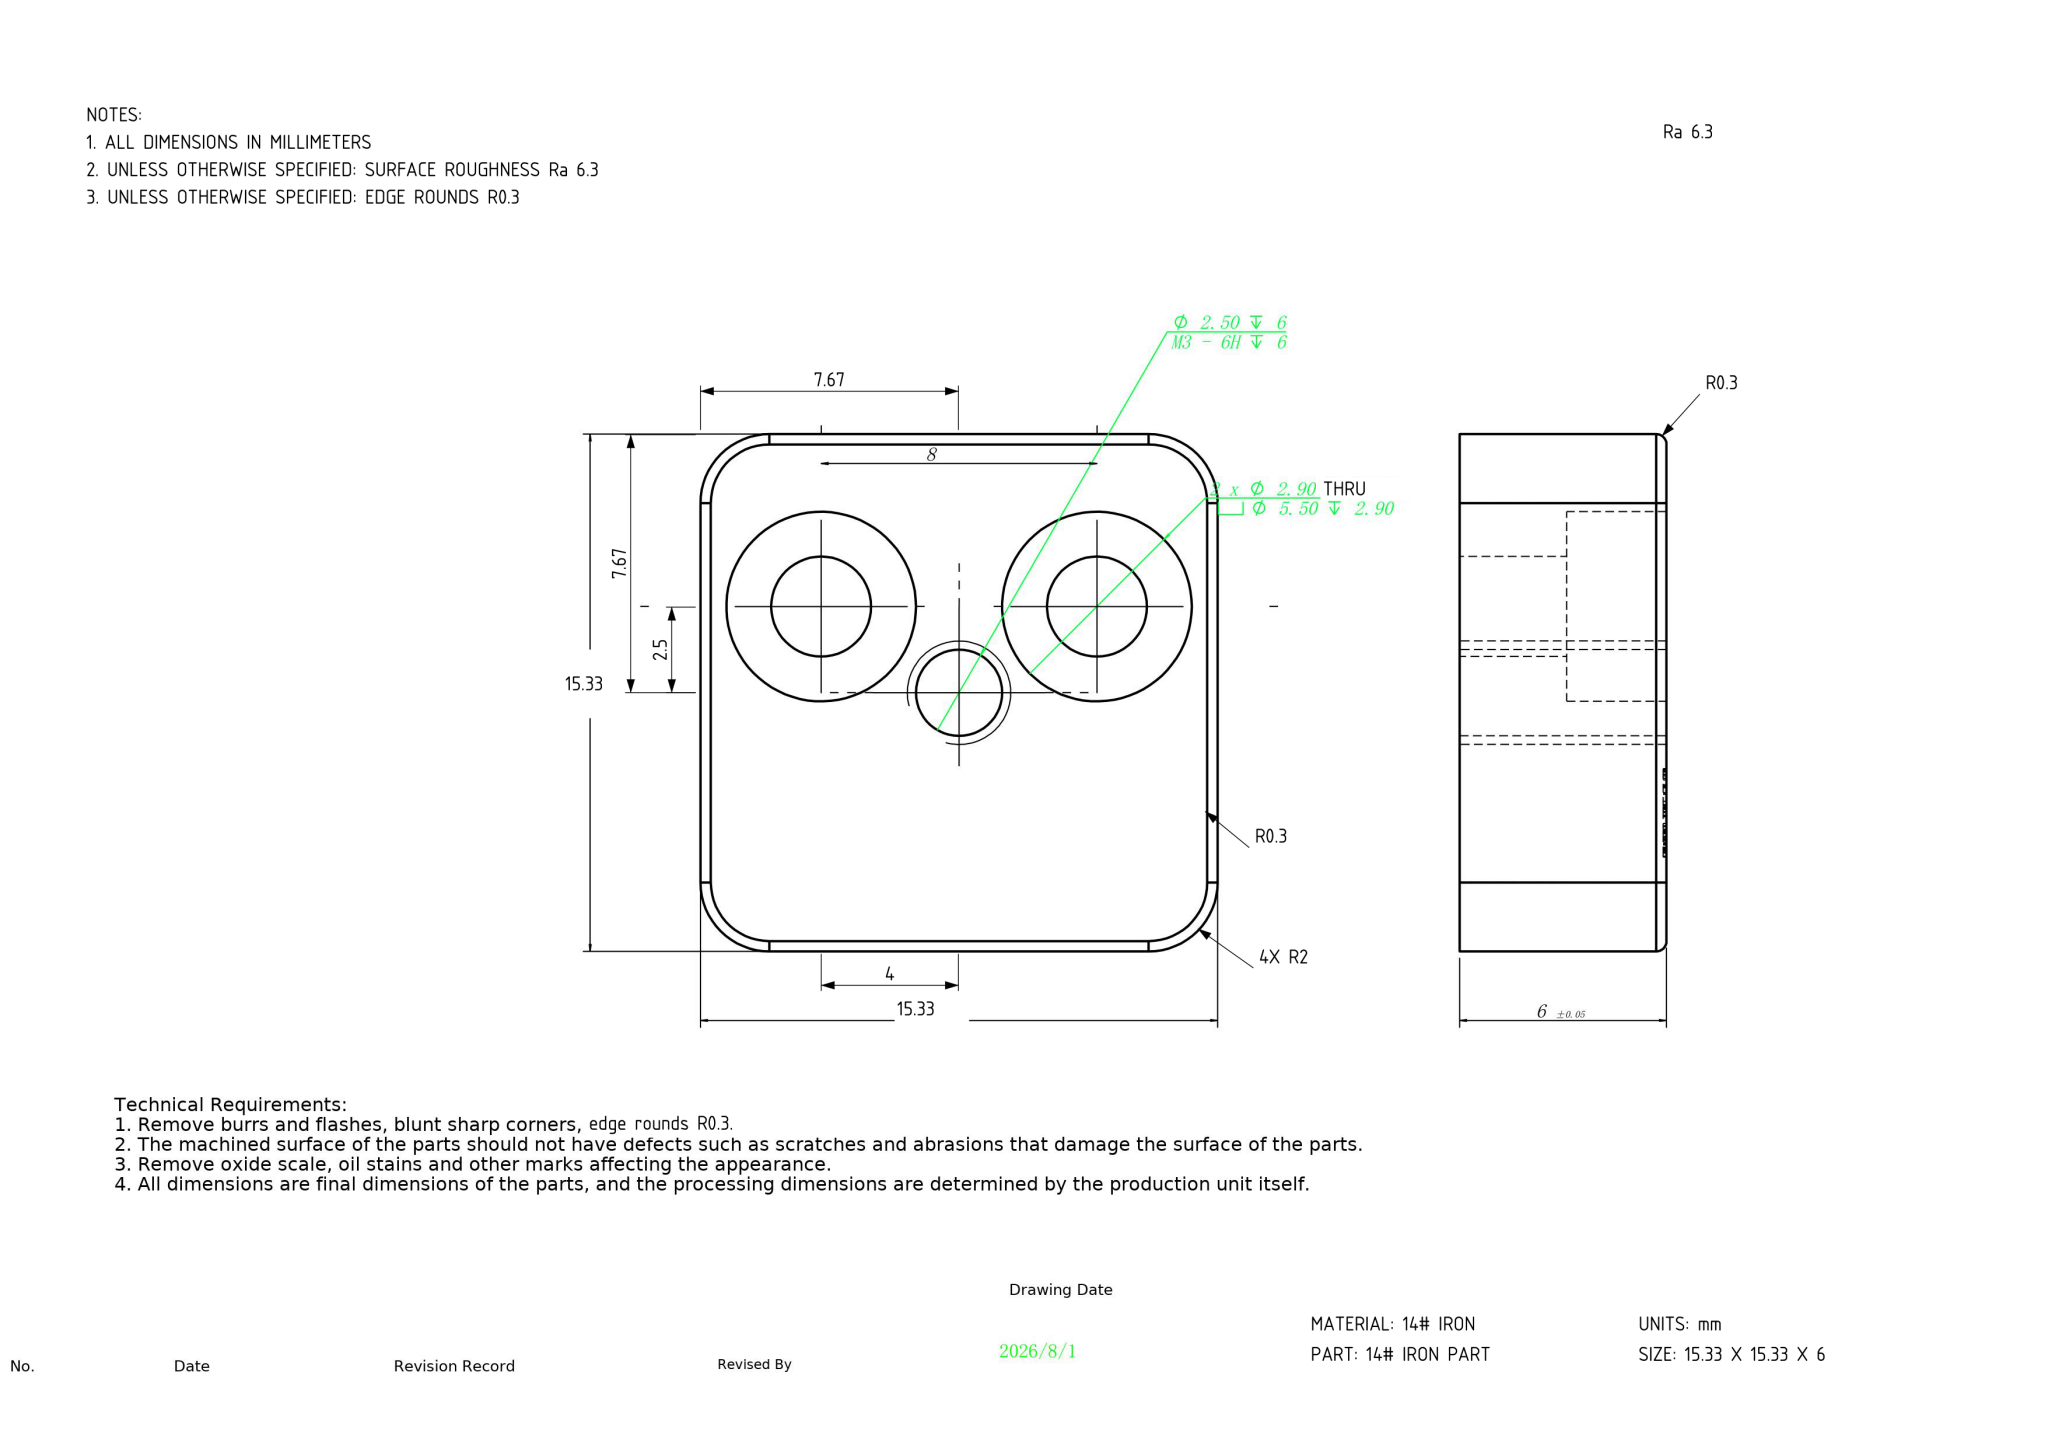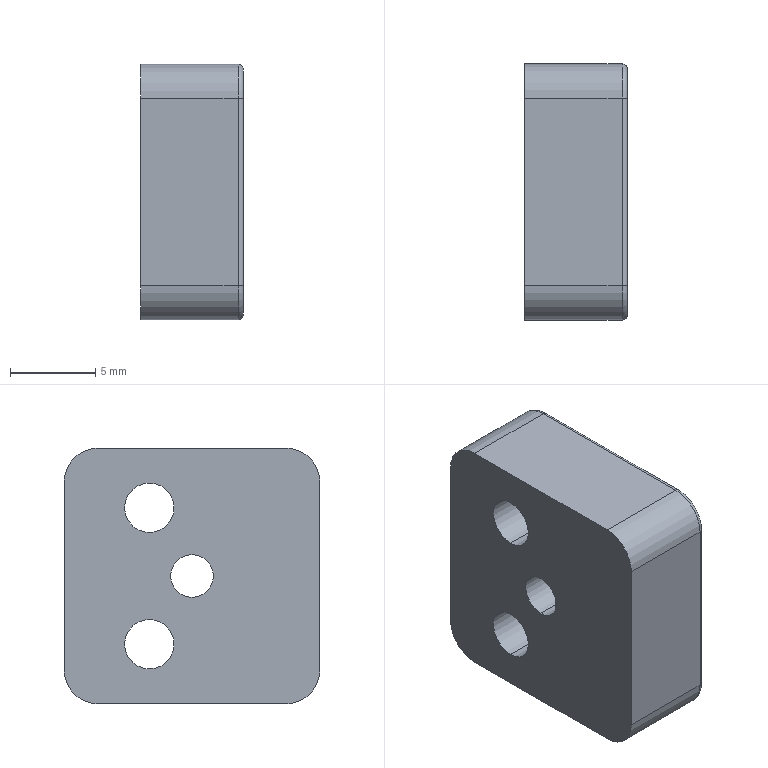Part | NX | mm | 1 solid | 165 faces | box 6 x 15 x 15 mm | volume 1120 mm3 | plane 112 | spline 31 | cylinder 18 | torus 4 | commonest cylinder face diameters 5.5 x4 2.9 x4 4 x4 0.6 x4 2.5 x2